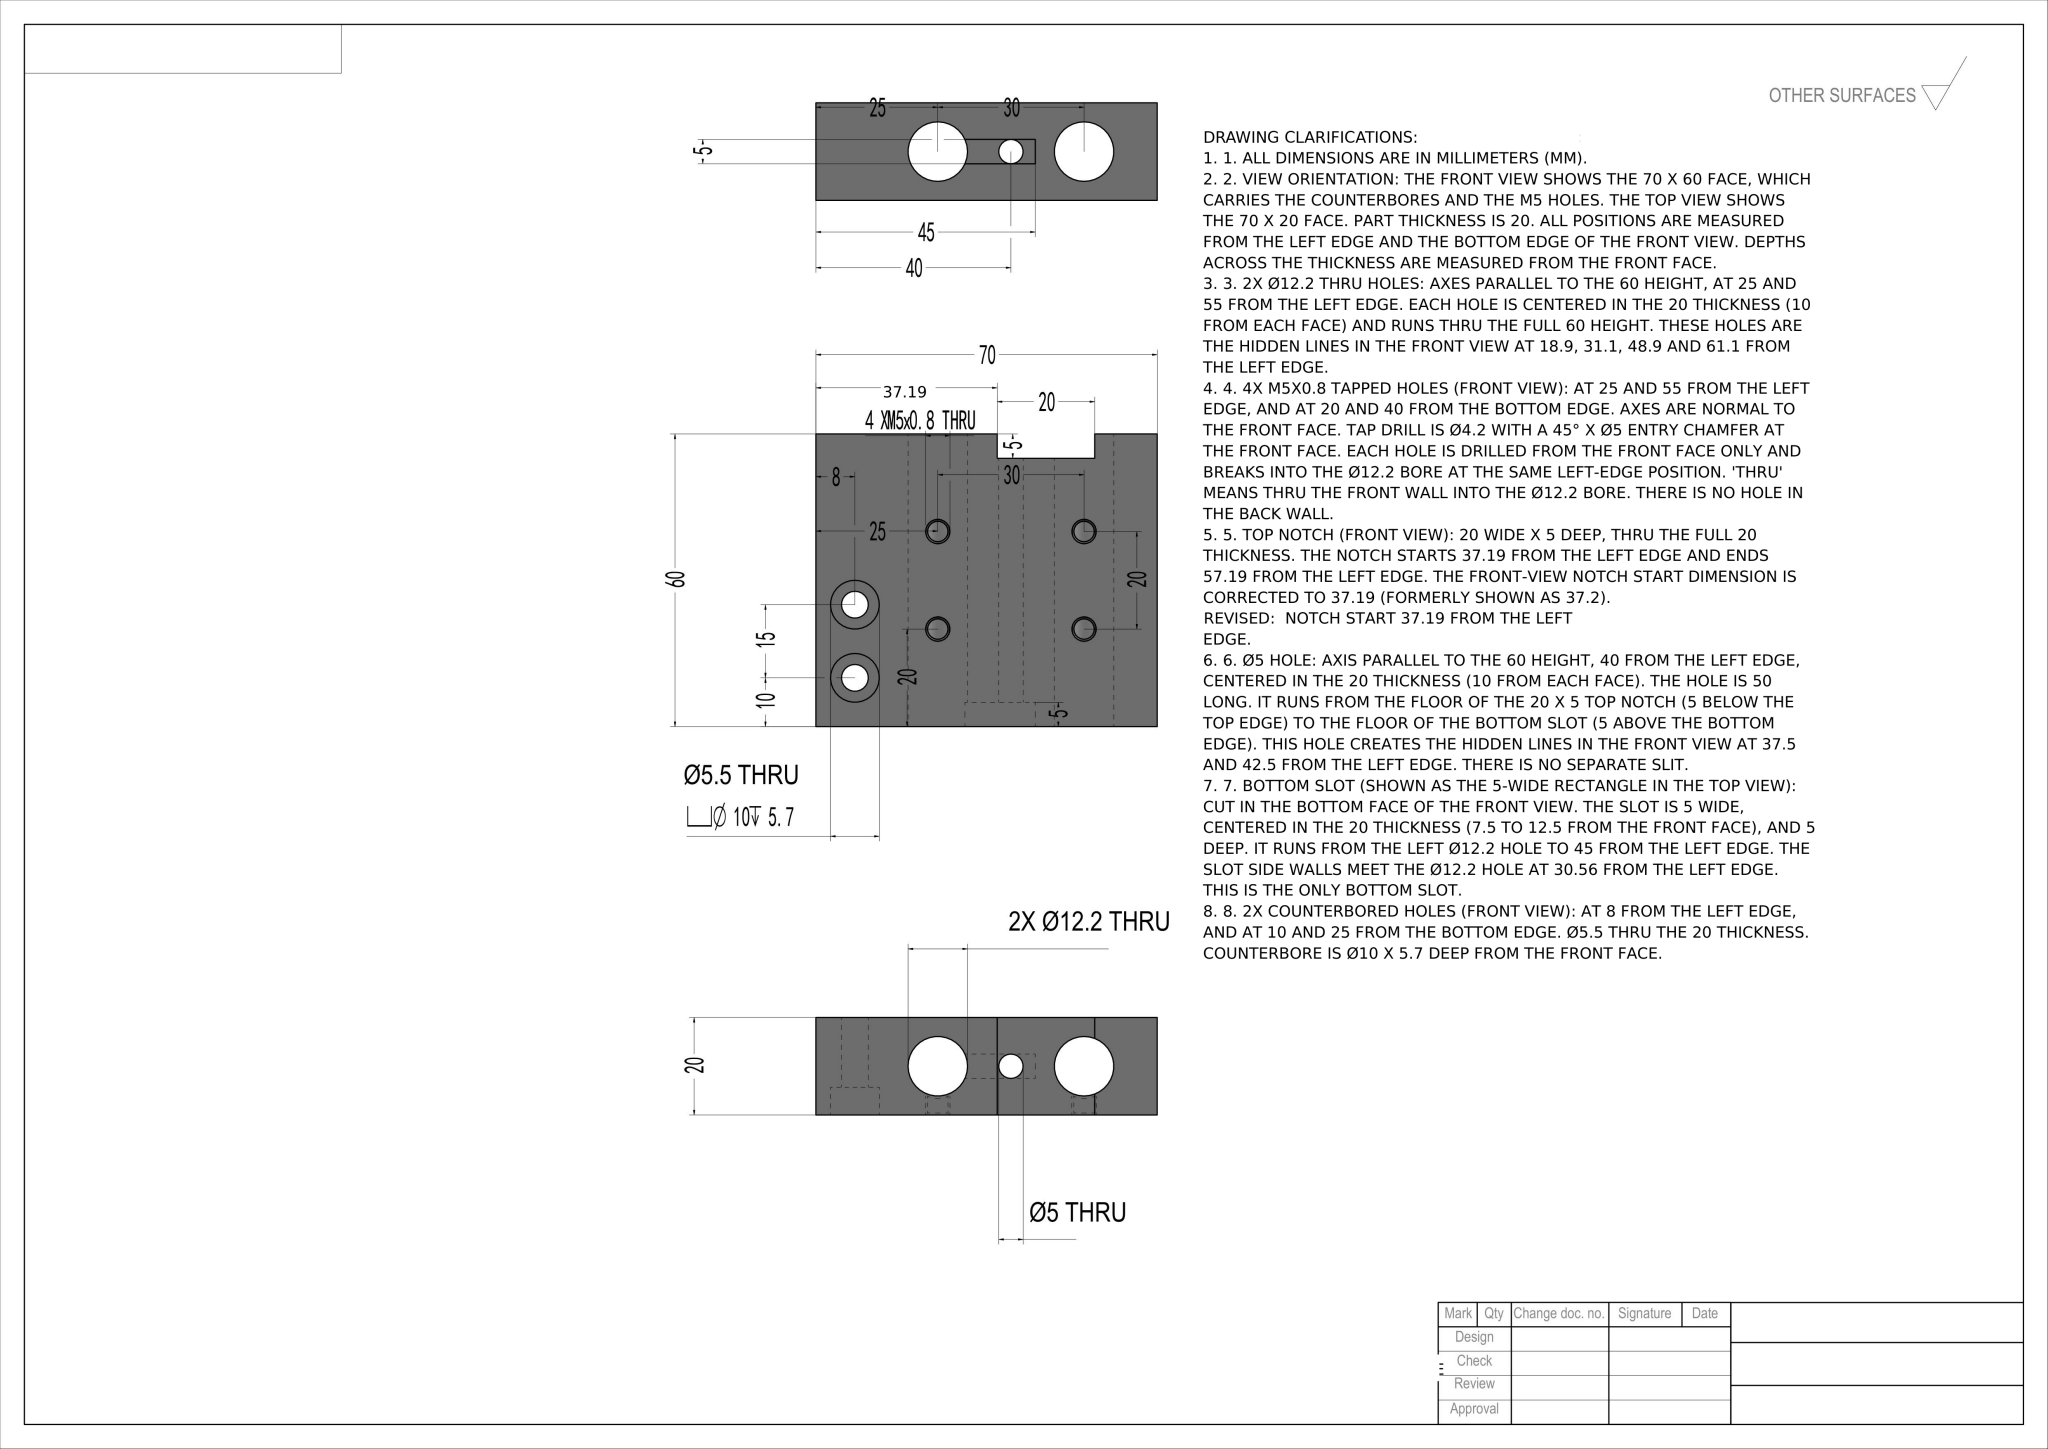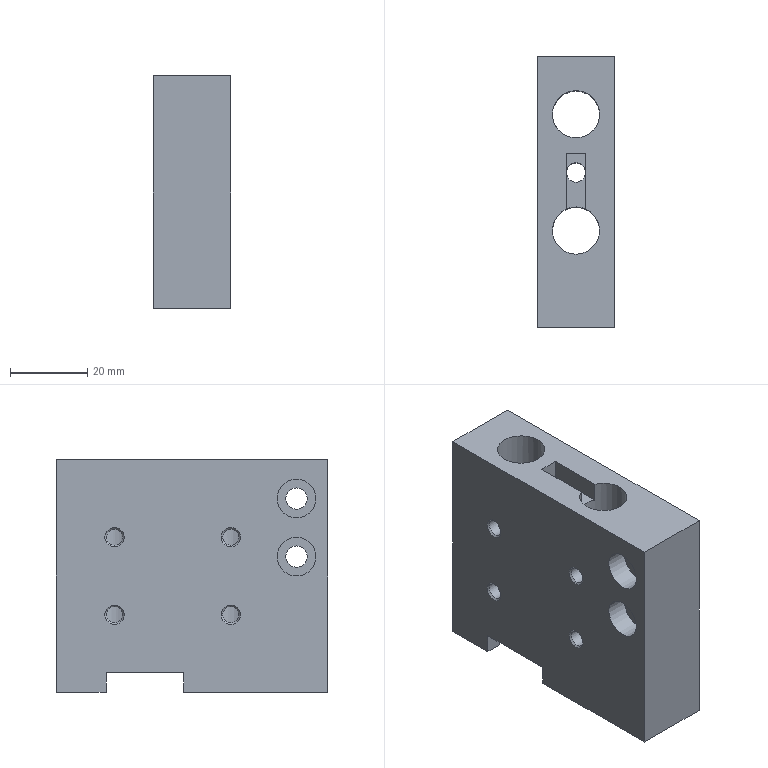Part | NX | mm | 1 solid | 37 faces | box 20 x 70 x 60 mm | volume 65256 mm3 | plane 18 | cylinder 11 | cone 4 | spline 4 | commonest cylinder face diameters 4.2 x4 5.5 x2 10 x2 12.2 x2 5 x1